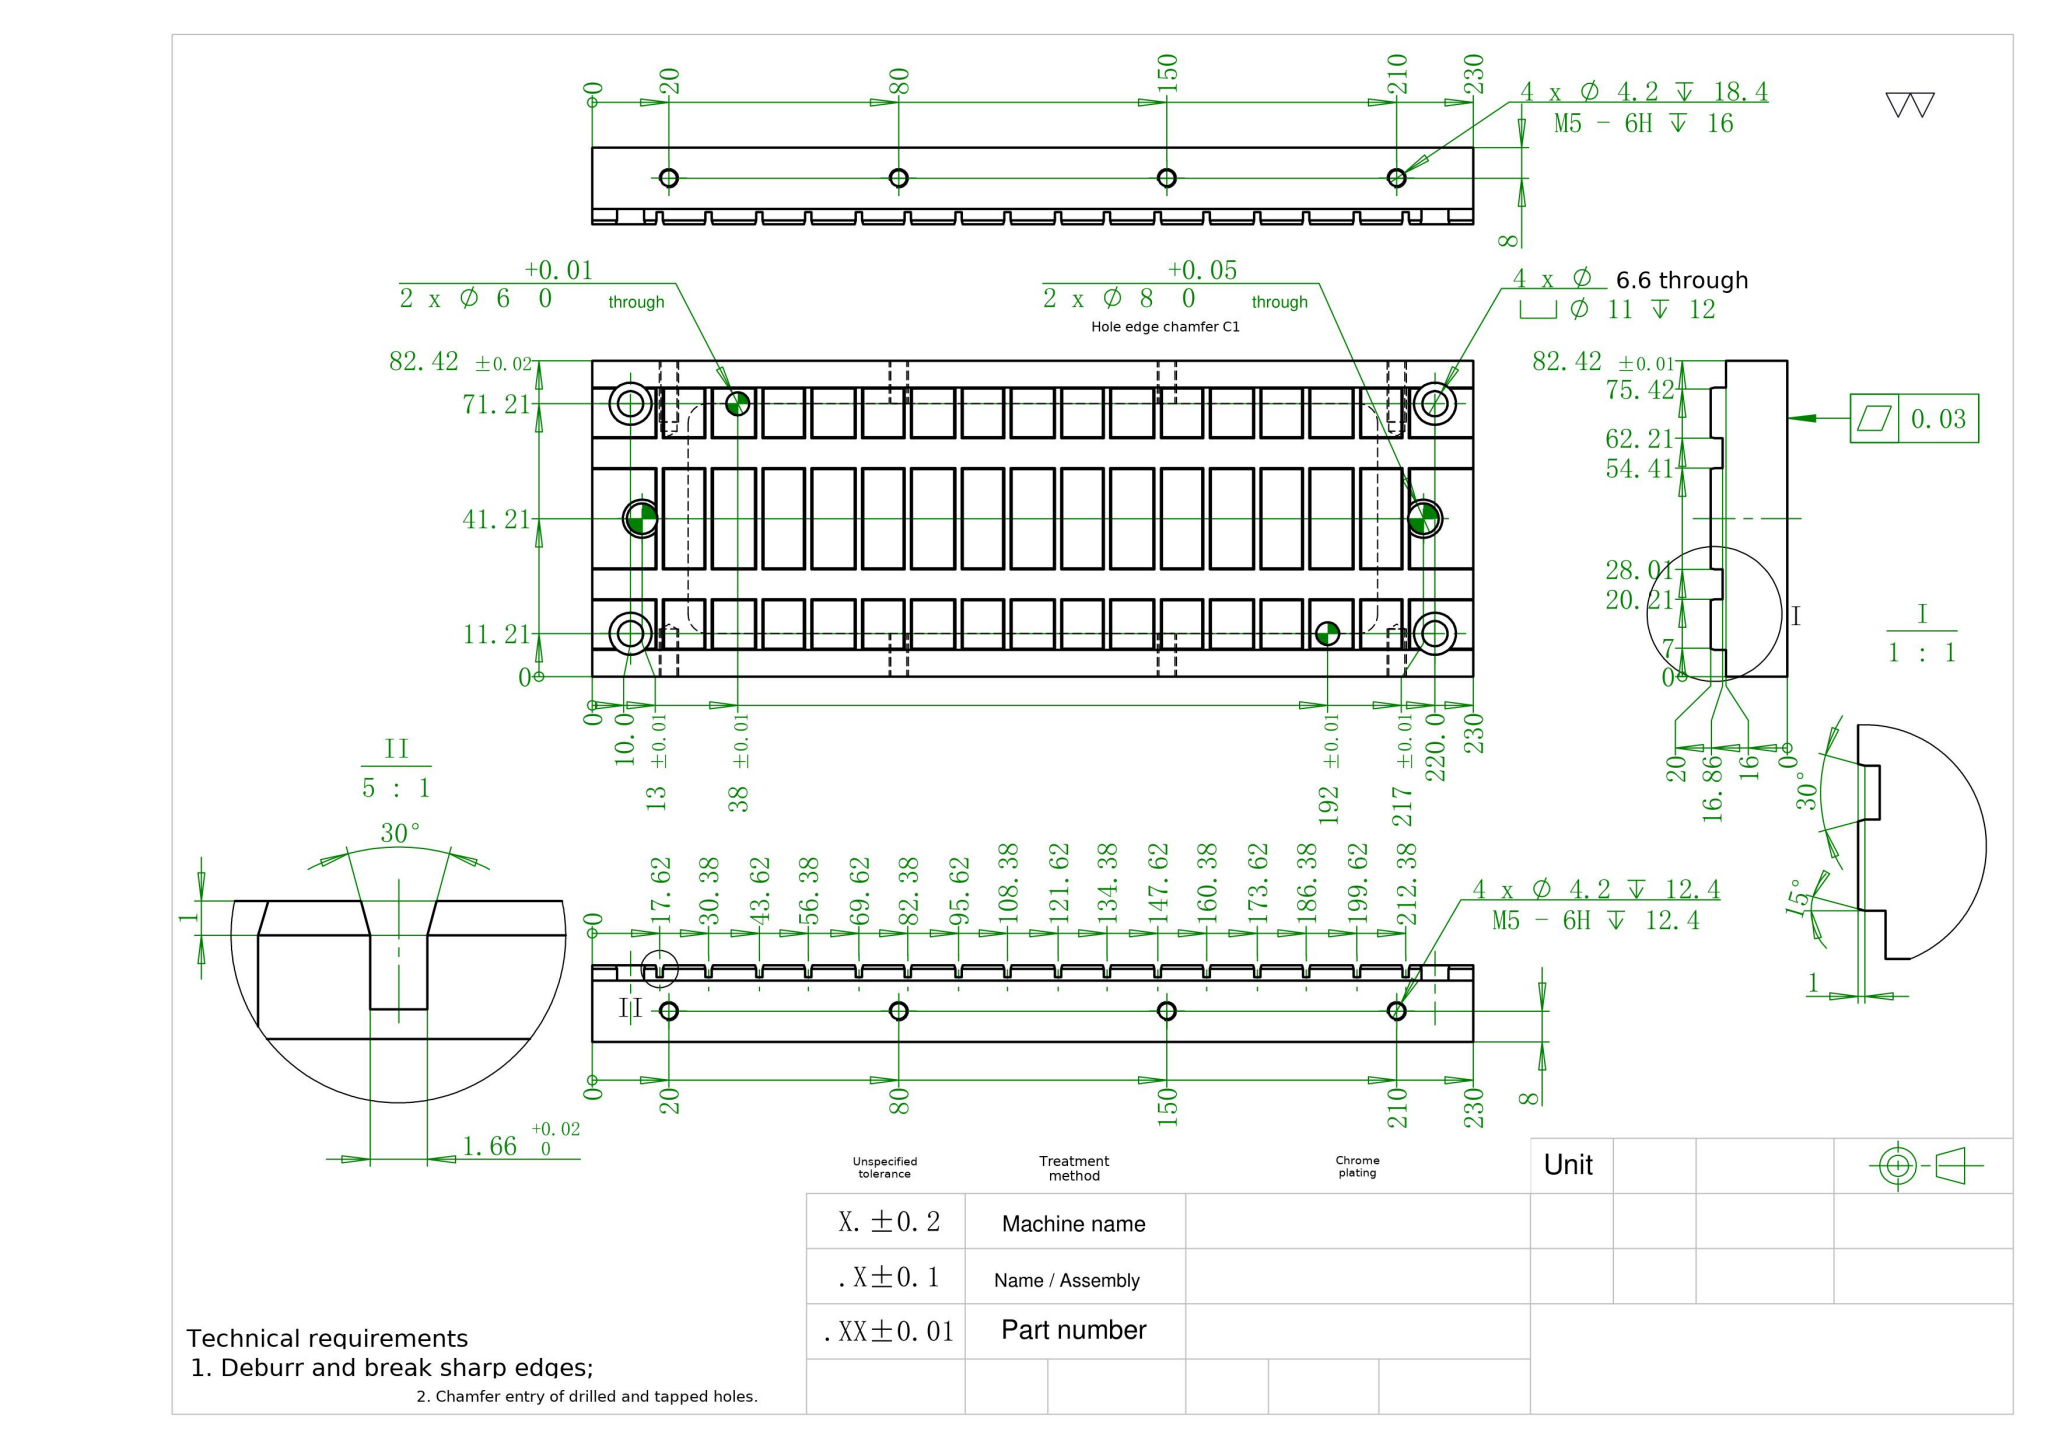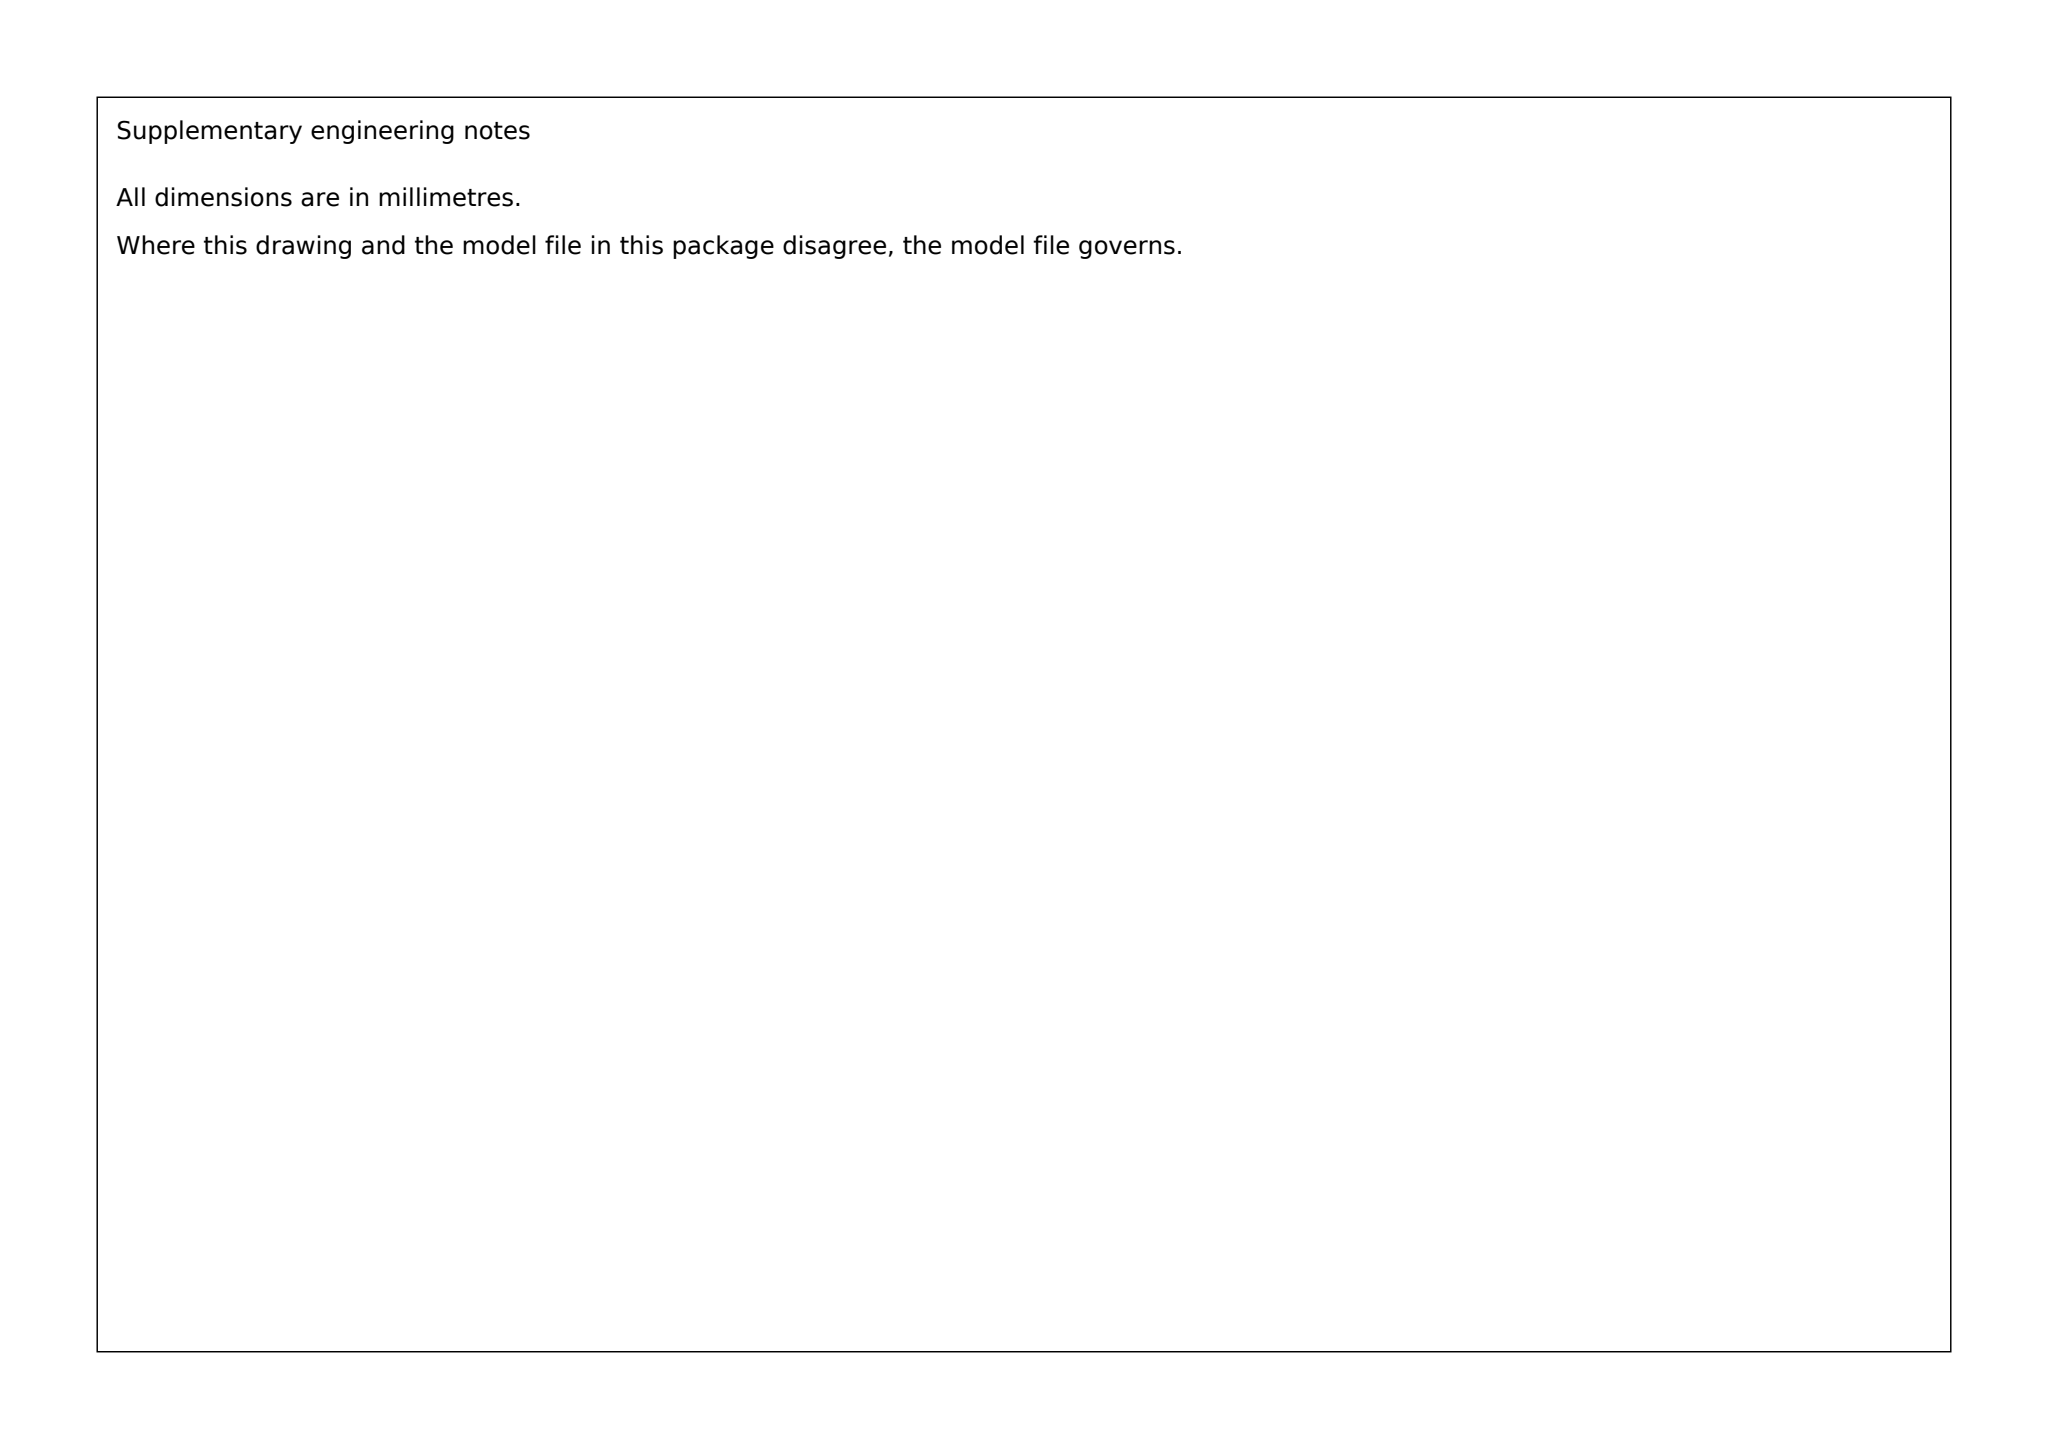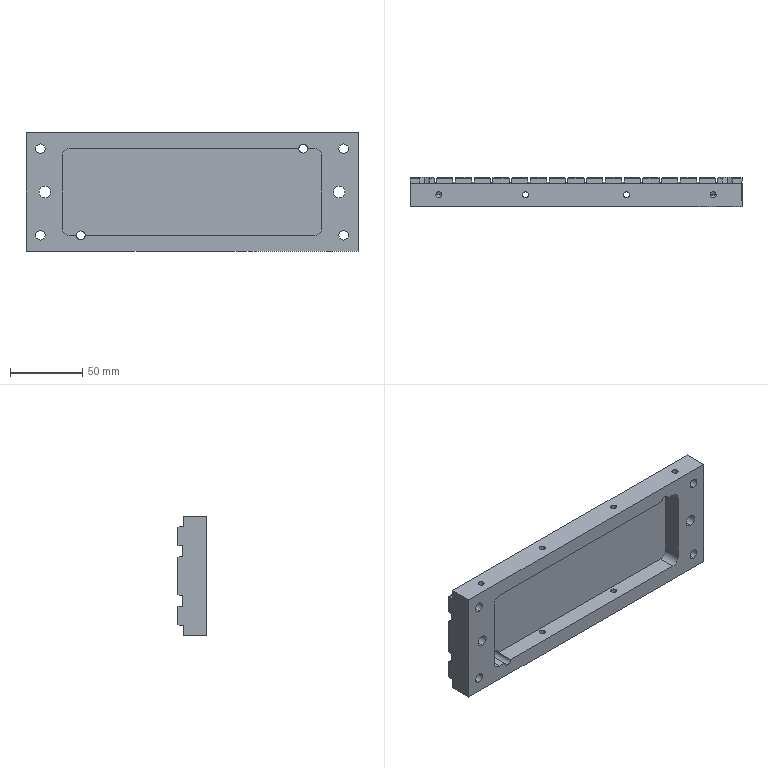Part | SolidWorks | mm | 1 solid | 504 faces | box 230 x 20 x 82.42 mm | volume 210981 mm3 | plane 446 | cylinder 44 | cone 14 | commonest cylinder face diameters 4.2 x16 6.6 x8 11 x8 8 x4 6 x4 10 x4